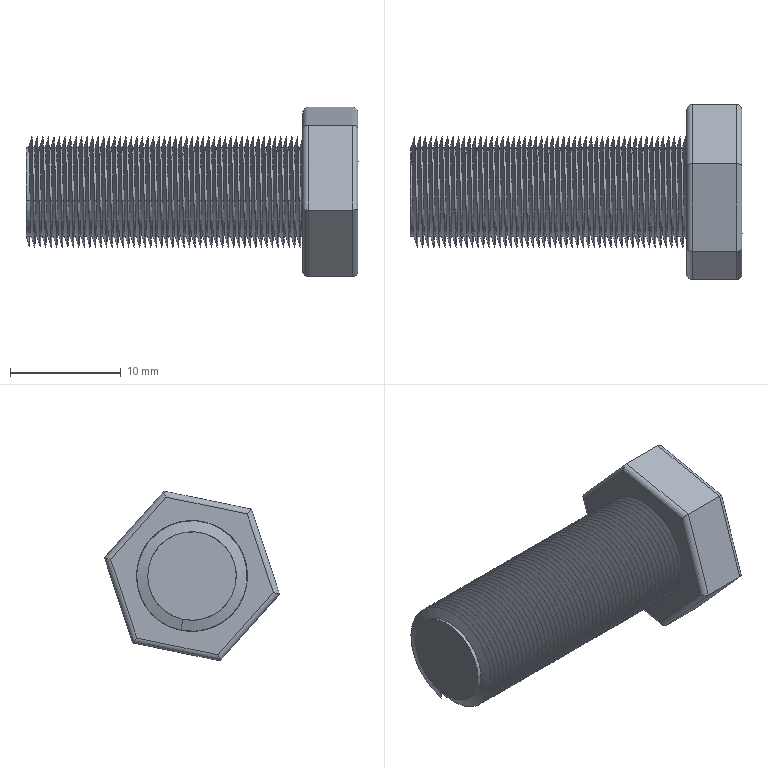Component | SolidWorks | CabinetFrameWeldmentDrawingPG50-01-00-1_BaseWeldingDrawingPG50-05-1_M10-30GroundingScrew-3 | 2 solids | 149 faces | volume 2219 mm3 | cylinder 136 | plane 11 | spline 2 | commonest cylinder face diameters 8 x122 1 x12 10 x2